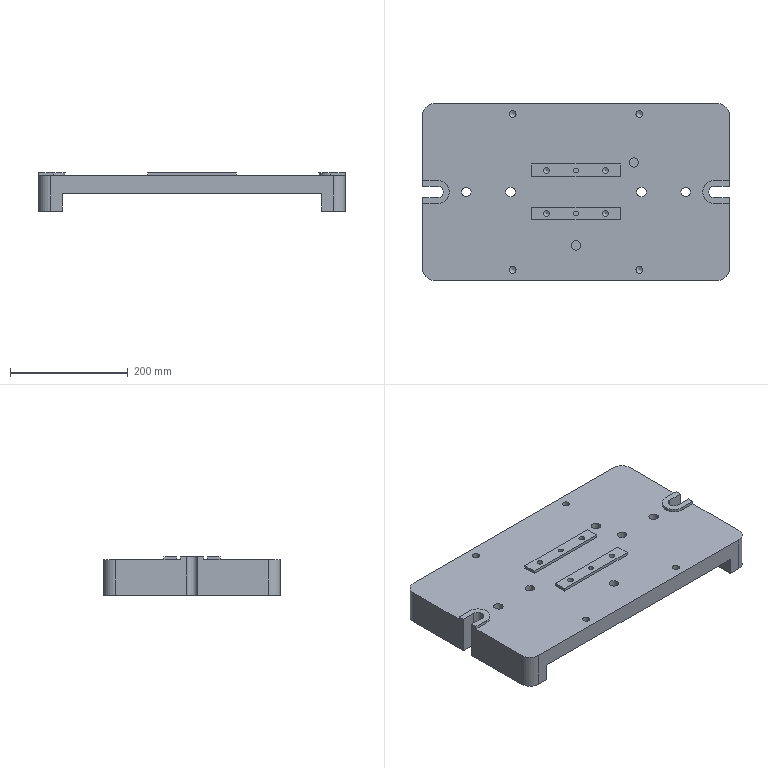Component | NX | FIXTURE_BODY | 1 solid | 68 faces | volume 5292013 mm3 | plane 36 | cylinder 24 | cone 8 | commonest cylinder face diameters 16 x6 40 x6 11.701 x4 9.732 x4 8 x2 20 x2